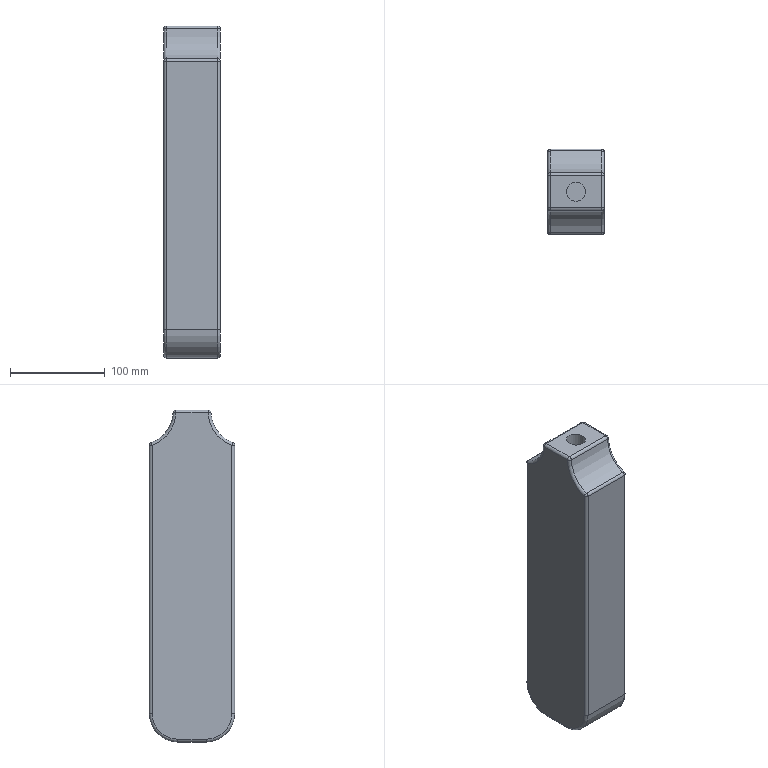Component | NX | HOUSING | 1 solid | 81 faces | volume 273146 mm3 | cylinder 36 | plane 29 | torus 8 | sphere 8 | commonest cylinder face diameters 6 x12 60 x3 30 x3 68.949 x2 25 x2 40 x2 10 x2 73.949 x2